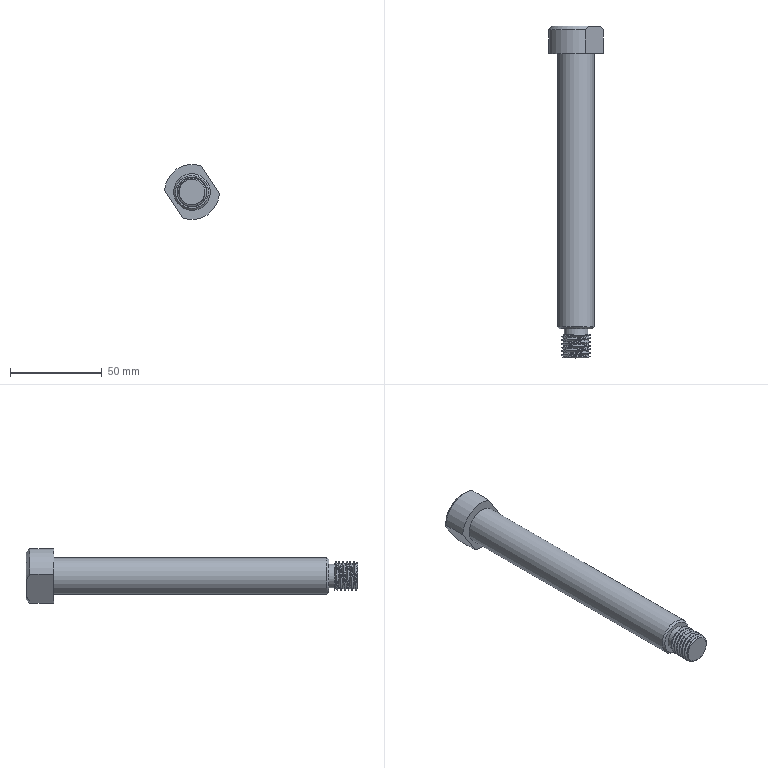Component | NX | LONG_PIN | 1 solid | 19 faces | volume 59136 mm3 | plane 7 | cylinder 6 | cone 4 | spline 2 | commonest cylinder face diameters 30 x2 20 x1 13 x1 16 x1 14 x1